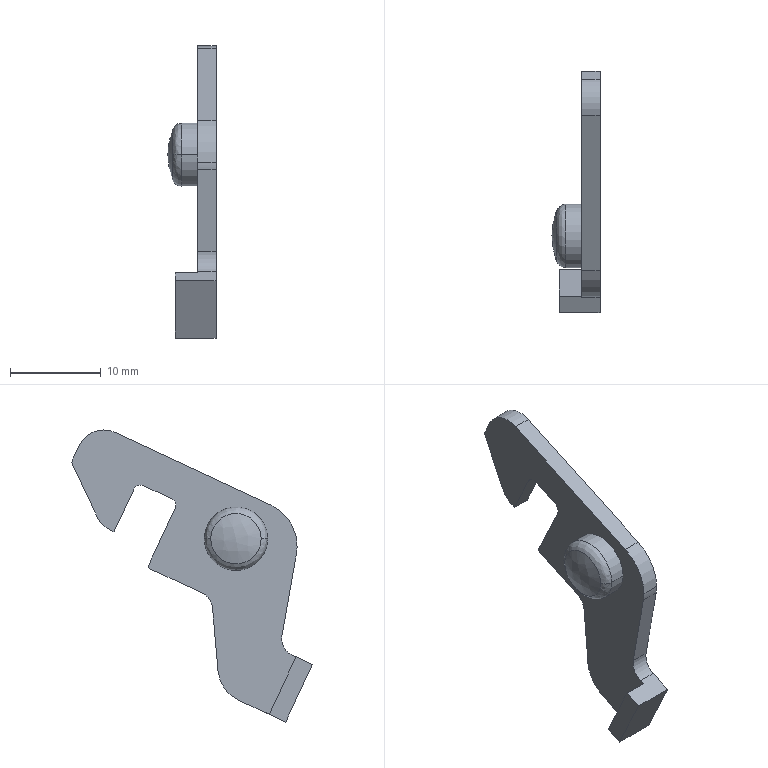Component | SolidWorks | RSDQA32-20DD-M9BL(0_0)-1_RSQ3220(0)-1 | 1 solid | 33 faces | box 5.3 x 26.56 x 32.2 mm | volume 826 mm3 | plane 17 | cylinder 13 | spline 3 | commonest cylinder face diameters 1.6 x3 10 x2 7 x2 6 x2 4 x2 8 x1 0.6 x1
STEP:
#1=COLOUR_RGB('',0.7922,0.8196,0.9333);
#2=FILL_AREA_STYLE_COLOUR('',#1);
#3=FILL_AREA_STYLE('',(#2));
#4=SURFACE_STYLE_FILL_AREA(#3);
#5=SURFACE_SIDE_STYLE('',(#4));
#6=SURFACE_STYLE_USAGE(.BOTH.,#5);
#7=PRESENTATION_STYLE_ASSIGNMENT((#6));
#8=CARTESIAN_POINT('',(0.0703,1.259,-0.6246));
#9=VERTEX_POINT('',#8);
#10=CARTESIAN_POINT('',(0.0703,0.9833,-0.6246));
#11=VERTEX_POINT('',#10);
#12=CARTESIAN_POINT('',(0.0703,1.121,-0.6246));
#13=DIRECTION('',(1.,0.,-0.));
#14=DIRECTION('',(0.,-1.,0.));
#15=AXIS2_PLACEMENT_3D('',#12,#13,#14);
#16=CIRCLE('',#15,0.1378);
#17=EDGE_CURVE('',#9,#11,#16,.T.);
#18=ORIENTED_EDGE('',*,*,#17,.F.);
#19=CARTESIAN_POINT('',(0.0297,1.231,-0.6246));
#20=VERTEX_POINT('',#19);
#21=CARTESIAN_POINT('',(0.0703,1.216,-0.6246));
#22=DIRECTION('',(0.,0.,1.));
#23=DIRECTION('',(0.,1.,0.));
#24=AXIS2_PLACEMENT_3D('',#21,#22,#23);
#25=CIRCLE('',#24,0.04331);
#26=EDGE_CURVE('',#9,#20,#25,.T.);
#27=ORIENTED_EDGE('',*,*,#26,.T.);
#28=CARTESIAN_POINT('',(0.0297,1.012,-0.6246));
#29=VERTEX_POINT('',#28);
#30=CARTESIAN_POINT('',(0.0297,1.121,-0.6246));
#31=DIRECTION('',(1.,0.,-0.));
#32=DIRECTION('',(0.,-1.,0.));
#33=AXIS2_PLACEMENT_3D('',#30,#31,#32);
#34=CIRCLE('',#33,0.1096);
#35=EDGE_CURVE('',#20,#29,#34,.T.);
#36=ORIENTED_EDGE('',*,*,#35,.T.);
#37=CARTESIAN_POINT('',(0.0703,1.027,-0.6246));
#38=DIRECTION('',(-0.,0.,-1.));
#39=DIRECTION('',(0.,-1.,0.));
#40=AXIS2_PLACEMENT_3D('',#37,#38,#39);
#41=CIRCLE('',#40,0.04331);
#42=EDGE_CURVE('',#11,#29,#41,.T.);
#43=ORIENTED_EDGE('',*,*,#42,.F.);
#44=EDGE_LOOP('',(#18,#27,#36,#43));
#45=FACE_OUTER_BOUND('',#44,.T.);
#46=CARTESIAN_POINT('',(0.0703,1.259,-0.6246));
#47=CARTESIAN_POINT('',(0.0703,1.259,-0.349));
#48=CARTESIAN_POINT('',(0.0703,0.9833,-0.349));
#49=CARTESIAN_POINT('',(0.0703,0.9833,-0.6246));
#50=CARTESIAN_POINT('',(0.05158,1.259,-0.6246));
#51=CARTESIAN_POINT('',(0.05158,1.259,-0.349));
#52=CARTESIAN_POINT('',(0.05158,0.9833,-0.349));
#53=CARTESIAN_POINT('',(0.05158,0.9833,-0.6246));
#54=CARTESIAN_POINT('',(0.03621,1.248,-0.6246));
#55=CARTESIAN_POINT('',(0.03621,1.248,-0.3704));
#56=CARTESIAN_POINT('',(0.03621,0.994,-0.3704));
#57=CARTESIAN_POINT('',(0.03621,0.994,-0.6246));
#58=CARTESIAN_POINT('',(0.0297,1.231,-0.6246));
#59=CARTESIAN_POINT('',(0.0297,1.231,-0.4055));
#60=CARTESIAN_POINT('',(0.0297,1.012,-0.4055));
#61=CARTESIAN_POINT('',(0.0297,1.012,-0.6246));
#62=(BOUNDED_SURFACE()B_SPLINE_SURFACE(3,3,((#46,#47,#48,#49),(#50,#51,#52,#53),(#54,#55,#56,#57),(#58,#59,#60,#61)),.UNSPECIFIED.,.F.,.F.,.F.)B_SPLINE_SURFACE_WITH_KNOTS((4,4),(4,4),(0.,1.),(0.,1.),.UNSPECIFIED.)GEOMETRIC_REPRESENTATION_ITEM()RATIONAL_B_SPLINE_SURFACE(((1.,0.3333,0.3333,1.),(0.8806,0.2935,0.2935,0.8806),(0.8806,0.2935,0.2935,0.8806),(1.,0.3333,0.3333,1.)))REPRESENTATION_ITEM('')SURFACE());
#63=ADVANCED_FACE('',(#45),#62,.T.);
#64=CARTESIAN_POINT('',(0.14,0.9696,-0.4781));
#65=VERTEX_POINT('',#64);
#66=CARTESIAN_POINT('',(0.14,0.8559,-0.6565));
#67=VERTEX_POINT('',#66);
#68=CARTESIAN_POINT('',(0.14,1.053,-0.6565));
#69=DIRECTION('',(1.,0.,-0.));
#70=DIRECTION('',(0.,-1.,0.));
#71=AXIS2_PLACEMENT_3D('',#68,#69,#70);
#72=CIRCLE('',#71,0.1969);
#73=EDGE_CURVE('',#65,#67,#72,.T.);
#74=ORIENTED_EDGE('',*,*,#73,.T.);
#75=CARTESIAN_POINT('',(0.2187,0.8559,-0.6565));
#76=VERTEX_POINT('',#75);
#77=CARTESIAN_POINT('',(0.14,0.8559,-0.6565));
#78=DIRECTION('',(1.,0.,-0.));
#79=VECTOR('',#78,39.37);
#80=LINE('',#77,#79);
#81=EDGE_CURVE('',#67,#76,#80,.T.);
#82=ORIENTED_EDGE('',*,*,#81,.T.);
#83=CARTESIAN_POINT('',(0.2187,0.9696,-0.4781));
#84=VERTEX_POINT('',#83);
#85=CARTESIAN_POINT('',(0.2187,1.053,-0.6565));
#86=DIRECTION('',(1.,0.,-0.));
#87=DIRECTION('',(0.,-1.,0.));
#88=AXIS2_PLACEMENT_3D('',#85,#86,#87);
#89=CIRCLE('',#88,0.1969);
#90=EDGE_CURVE('',#84,#76,#89,.T.);
#91=ORIENTED_EDGE('',*,*,#90,.F.);
#92=CARTESIAN_POINT('',(0.14,0.9696,-0.4781));
#93=DIRECTION('',(-1.,-0.,0.));
#94=VECTOR('',#93,39.37);
#95=LINE('',#92,#94);
#96=EDGE_CURVE('',#84,#65,#95,.T.);
#97=ORIENTED_EDGE('',*,*,#96,.T.);
#98=EDGE_LOOP('',(#74,#82,#91,#97));
#99=FACE_OUTER_BOUND('',#98,.T.);
#100=CARTESIAN_POINT('',(0.14,1.053,-0.6565));
#101=DIRECTION('',(1.,0.,-0.));
#102=DIRECTION('',(0.,-1.,0.));
#103=AXIS2_PLACEMENT_3D('',#100,#101,#102);
#104=CYLINDRICAL_SURFACE('',#103,0.1969);
#105=ADVANCED_FACE('',(#99),#104,.T.);
#106=CARTESIAN_POINT('',(0.14,1.385,-0.4927));
#107=VERTEX_POINT('',#106);
#108=CARTESIAN_POINT('',(0.14,1.382,-0.4794));
#109=VERTEX_POINT('',#108);
#110=CARTESIAN_POINT('',(0.14,1.414,-0.4794));
#111=DIRECTION('',(-1.,-0.,0.));
#112=DIRECTION('',(0.,-1.,0.));
#113=AXIS2_PLACEMENT_3D('',#110,#111,#112);
#114=CIRCLE('',#113,0.0315);
#115=EDGE_CURVE('',#107,#109,#114,.T.);
#116=ORIENTED_EDGE('',*,*,#115,.T.);
#117=CARTESIAN_POINT('',(0.2187,1.382,-0.4794));
#118=VERTEX_POINT('',#117);
#119=CARTESIAN_POINT('',(0.14,1.382,-0.4794));
#120=DIRECTION('',(1.,0.,-0.));
#121=VECTOR('',#120,39.37);
#122=LINE('',#119,#121);
#123=EDGE_CURVE('',#109,#118,#122,.T.);
#124=ORIENTED_EDGE('',*,*,#123,.T.);
#125=CARTESIAN_POINT('',(0.2187,1.385,-0.4927));
#126=VERTEX_POINT('',#125);
#127=CARTESIAN_POINT('',(0.2187,1.414,-0.4794));
#128=DIRECTION('',(1.,0.,-0.));
#129=DIRECTION('',(0.,-1.,0.));
#130=AXIS2_PLACEMENT_3D('',#127,#128,#129);
#131=CIRCLE('',#130,0.0315);
#132=EDGE_CURVE('',#118,#126,#131,.T.);
#133=ORIENTED_EDGE('',*,*,#132,.T.);
#134=CARTESIAN_POINT('',(0.14,1.385,-0.4927));
#135=DIRECTION('',(1.,0.,-0.));
#136=VECTOR('',#135,39.37);
#137=LINE('',#134,#136);
#138=EDGE_CURVE('',#107,#126,#137,.T.);
#139=ORIENTED_EDGE('',*,*,#138,.F.);
#140=EDGE_LOOP('',(#116,#124,#133,#139));
#141=FACE_OUTER_BOUND('',#140,.T.);
#142=CARTESIAN_POINT('',(0.14,1.414,-0.4794));
#143=DIRECTION('',(1.,0.,-0.));
#144=DIRECTION('',(0.,-1.,0.));
#145=AXIS2_PLACEMENT_3D('',#142,#143,#144);
#146=CYLINDRICAL_SURFACE('',#145,0.0315);
#147=ADVANCED_FACE('',(#141),#146,.F.);
#148=CARTESIAN_POINT('',(0.0703,1.121,-0.6246));
#149=DIRECTION('',(1.,0.,-0.));
#150=DIRECTION('',(0.,-1.,0.));
#151=AXIS2_PLACEMENT_3D('',#148,#149,#150);
#152=CIRCLE('',#151,0.1378);
#153=EDGE_CURVE('',#11,#9,#152,.T.);
#154=ORIENTED_EDGE('',*,*,#153,.T.);
#155=CARTESIAN_POINT('',(0.14,1.259,-0.6246));
#156=VERTEX_POINT('',#155);
#157=CARTESIAN_POINT('',(0.1051,1.259,-0.6246));
#158=DIRECTION('',(1.,0.,-0.));
#159=VECTOR('',#158,39.37);
#160=LINE('',#157,#159);
#161=EDGE_CURVE('',#9,#156,#160,.T.);
#162=ORIENTED_EDGE('',*,*,#161,.T.);
#163=CARTESIAN_POINT('',(0.14,0.9833,-0.6246));
#164=VERTEX_POINT('',#163);
#165=CARTESIAN_POINT('',(0.14,1.121,-0.6246));
#166=DIRECTION('',(-1.,-0.,0.));
#167=DIRECTION('',(0.,-1.,0.));
#168=AXIS2_PLACEMENT_3D('',#165,#166,#167);
#169=CIRCLE('',#168,0.1378);
#170=EDGE_CURVE('',#156,#164,#169,.T.);
#171=ORIENTED_EDGE('',*,*,#170,.T.);
#172=CARTESIAN_POINT('',(0.1051,0.9833,-0.6246));
#173=DIRECTION('',(1.,0.,-0.));
#174=VECTOR('',#173,39.37);
#175=LINE('',#172,#174);
#176=EDGE_CURVE('',#11,#164,#175,.T.);
#177=ORIENTED_EDGE('',*,*,#176,.F.);
#178=EDGE_LOOP('',(#154,#162,#171,#177));
#179=FACE_OUTER_BOUND('',#178,.T.);
#180=CARTESIAN_POINT('',(0.1051,1.121,-0.6246));
#181=DIRECTION('',(1.,0.,-0.));
#182=DIRECTION('',(0.,-1.,0.));
#183=AXIS2_PLACEMENT_3D('',#180,#181,#182);
#184=CYLINDRICAL_SURFACE('',#183,0.1378);
#185=ADVANCED_FACE('',(#179),#184,.T.);
#186=CARTESIAN_POINT('',(0.2187,1.666,-0.5876));
#187=VERTEX_POINT('',#186);
#188=CARTESIAN_POINT('',(0.2187,1.65,-0.5951));
#189=VERTEX_POINT('',#188);
#190=CARTESIAN_POINT('',(0.2187,1.666,-0.5876));
#191=DIRECTION('',(-0.,-0.9063,-0.4226));
#192=VECTOR('',#191,39.37);
#193=LINE('',#190,#192);
#194=EDGE_CURVE('',#187,#189,#193,.T.);
#195=ORIENTED_EDGE('',*,*,#194,.F.);
#196=CARTESIAN_POINT('',(0.2187,1.723,-0.5305));
#197=VERTEX_POINT('',#196);
#198=CARTESIAN_POINT('',(0.2187,1.616,-0.4806));
#199=DIRECTION('',(1.,0.,-0.));
#200=DIRECTION('',(0.,-1.,0.));
#201=AXIS2_PLACEMENT_3D('',#198,#199,#200);
#202=CIRCLE('',#201,0.1181);
#203=EDGE_CURVE('',#187,#197,#202,.T.);
#204=ORIENTED_EDGE('',*,*,#203,.T.);
#205=CARTESIAN_POINT('',(0.2187,1.835,-0.2918));
#206=VERTEX_POINT('',#205);
#207=CARTESIAN_POINT('',(0.2187,1.723,-0.5305));
#208=DIRECTION('',(0.,0.4226,0.9063));
#209=VECTOR('',#208,39.37);
#210=LINE('',#207,#209);
#211=EDGE_CURVE('',#197,#206,#210,.T.);
#212=ORIENTED_EDGE('',*,*,#211,.T.);
#213=CARTESIAN_POINT('',(0.2187,1.801,-0.2205));
#214=VERTEX_POINT('',#213);
#215=CARTESIAN_POINT('',(0.2187,1.835,-0.2918));
#216=DIRECTION('',(0.,-0.4226,0.9063));
#217=VECTOR('',#216,39.37);
#218=LINE('',#215,#217);
#219=EDGE_CURVE('',#206,#214,#218,.T.);
#220=ORIENTED_EDGE('',*,*,#219,.T.);
#221=CARTESIAN_POINT('',(0.2187,1.644,-0.1634));
#222=VERTEX_POINT('',#221);
#223=CARTESIAN_POINT('',(0.2187,1.694,-0.2704));
#224=DIRECTION('',(1.,0.,-0.));
#225=DIRECTION('',(0.,-1.,0.));
#226=AXIS2_PLACEMENT_3D('',#223,#224,#225);
#227=CIRCLE('',#226,0.1181);
#228=EDGE_CURVE('',#214,#222,#227,.T.);
#229=ORIENTED_EDGE('',*,*,#228,.T.);
#230=CARTESIAN_POINT('',(0.2187,1.644,-0.1634));
#231=DIRECTION('',(-0.,-0.9063,-0.4226));
#232=VECTOR('',#231,39.37);
#233=LINE('',#230,#232);
#234=EDGE_CURVE('',#222,#84,#233,.T.);
#235=ORIENTED_EDGE('',*,*,#234,.T.);
#236=ORIENTED_EDGE('',*,*,#90,.T.);
#237=CARTESIAN_POINT('',(0.2187,0.8589,-0.6907));
#238=VERTEX_POINT('',#237);
#239=CARTESIAN_POINT('',(0.2187,1.053,-0.6565));
#240=DIRECTION('',(1.,0.,-0.));
#241=DIRECTION('',(0.,-1.,0.));
#242=AXIS2_PLACEMENT_3D('',#239,#240,#241);
#243=CIRCLE('',#242,0.1969);
#244=EDGE_CURVE('',#76,#238,#243,.T.);
#245=ORIENTED_EDGE('',*,*,#244,.T.);
#246=CARTESIAN_POINT('',(0.2187,0.9213,-1.044));
#247=VERTEX_POINT('',#246);
#248=CARTESIAN_POINT('',(0.2187,0.8589,-0.6907));
#249=DIRECTION('',(-0.,0.1736,-0.9848));
#250=VECTOR('',#249,39.37);
#251=LINE('',#248,#250);
#252=EDGE_CURVE('',#238,#247,#251,.T.);
#253=ORIENTED_EDGE('',*,*,#252,.T.);
#254=CARTESIAN_POINT('',(0.2187,0.877,-1.129));
#255=VERTEX_POINT('',#254);
#256=CARTESIAN_POINT('',(0.2187,0.8438,-1.058));
#257=DIRECTION('',(-1.,-0.,0.));
#258=DIRECTION('',(0.,-1.,-0.));
#259=AXIS2_PLACEMENT_3D('',#256,#257,#258);
#260=CIRCLE('',#259,0.07874);
#261=EDGE_CURVE('',#247,#255,#260,.T.);
#262=ORIENTED_EDGE('',*,*,#261,.T.);
#263=CARTESIAN_POINT('',(0.2187,0.7891,-1.17));
#264=VERTEX_POINT('',#263);
#265=CARTESIAN_POINT('',(0.2187,0.877,-1.129));
#266=DIRECTION('',(-0.,-0.9063,-0.4226));
#267=VECTOR('',#266,39.37);
#268=LINE('',#265,#267);
#269=EDGE_CURVE('',#255,#264,#268,.T.);
#270=ORIENTED_EDGE('',*,*,#269,.T.);
#271=CARTESIAN_POINT('',(0.2187,0.9056,-1.42));
#272=VERTEX_POINT('',#271);
#273=CARTESIAN_POINT('',(0.2187,0.7891,-1.17));
#274=DIRECTION('',(-0.,0.4226,-0.9063));
#275=VECTOR('',#274,39.37);
#276=LINE('',#273,#275);
#277=EDGE_CURVE('',#264,#272,#276,.T.);
#278=ORIENTED_EDGE('',*,*,#277,.T.);
#279=CARTESIAN_POINT('',(0.2187,1.109,-1.325));
#280=VERTEX_POINT('',#279);
#281=CARTESIAN_POINT('',(0.2187,0.9056,-1.42));
#282=DIRECTION('',(0.,0.9063,0.4226));
#283=VECTOR('',#282,39.37);
#284=LINE('',#281,#283);
#285=EDGE_CURVE('',#272,#280,#284,.T.);
#286=ORIENTED_EDGE('',*,*,#285,.T.);
#287=CARTESIAN_POINT('',(0.2187,1.199,-1.196));
#288=VERTEX_POINT('',#287);
#289=CARTESIAN_POINT('',(0.2187,1.042,-1.183));
#290=DIRECTION('',(1.,0.,-0.));
#291=DIRECTION('',(0.,-1.,0.));
#292=AXIS2_PLACEMENT_3D('',#289,#290,#291);
#293=CIRCLE('',#292,0.1575);
#294=EDGE_CURVE('',#280,#288,#293,.T.);
#295=ORIENTED_EDGE('',*,*,#294,.T.);
#296=CARTESIAN_POINT('',(0.2187,1.223,-0.9247));
#297=VERTEX_POINT('',#296);
#298=CARTESIAN_POINT('',(0.2187,1.199,-1.196));
#299=DIRECTION('',(0.,0.08716,0.9962));
#300=VECTOR('',#299,39.37);
#301=LINE('',#298,#300);
#302=EDGE_CURVE('',#288,#297,#301,.T.);
#303=ORIENTED_EDGE('',*,*,#302,.T.);
#304=CARTESIAN_POINT('',(0.2187,1.268,-0.8602));
#305=VERTEX_POINT('',#304);
#306=CARTESIAN_POINT('',(0.2187,1.301,-0.9316));
#307=DIRECTION('',(-1.,-0.,0.));
#308=DIRECTION('',(0.,-1.,0.));
#309=AXIS2_PLACEMENT_3D('',#306,#307,#308);
#310=CIRCLE('',#309,0.07874);
#311=EDGE_CURVE('',#297,#305,#310,.T.);
#312=ORIENTED_EDGE('',*,*,#311,.T.);
#313=CARTESIAN_POINT('',(0.2187,1.494,-0.7546));
#314=VERTEX_POINT('',#313);
#315=CARTESIAN_POINT('',(0.2187,1.268,-0.8602));
#316=DIRECTION('',(0.,0.9063,0.4226));
#317=VECTOR('',#316,39.37);
#318=LINE('',#315,#317);
#319=EDGE_CURVE('',#305,#314,#318,.T.);
#320=ORIENTED_EDGE('',*,*,#319,.T.);
#321=CARTESIAN_POINT('',(0.2187,1.5,-0.7389));
#322=VERTEX_POINT('',#321);
#323=CARTESIAN_POINT('',(0.2187,1.489,-0.7439));
#324=DIRECTION('',(-1.,-0.,0.));
#325=DIRECTION('',(0.,-1.,0.));
#326=AXIS2_PLACEMENT_3D('',#323,#324,#325);
#327=CIRCLE('',#326,0.01181);
#328=EDGE_CURVE('',#322,#314,#327,.T.);
#329=ORIENTED_EDGE('',*,*,#328,.F.);
#330=CARTESIAN_POINT('',(0.2187,1.5,-0.7389));
#331=DIRECTION('',(0.,-0.4226,0.9063));
#332=VECTOR('',#331,39.37);
#333=LINE('',#330,#332);
#334=EDGE_CURVE('',#322,#126,#333,.T.);
#335=ORIENTED_EDGE('',*,*,#334,.T.);
#336=ORIENTED_EDGE('',*,*,#132,.F.);
#337=CARTESIAN_POINT('',(0.2187,1.401,-0.4509));
#338=VERTEX_POINT('',#337);
#339=CARTESIAN_POINT('',(0.2187,1.414,-0.4794));
#340=DIRECTION('',(1.,0.,-0.));
#341=DIRECTION('',(0.,-1.,0.));
#342=AXIS2_PLACEMENT_3D('',#339,#340,#341);
#343=CIRCLE('',#342,0.0315);
#344=EDGE_CURVE('',#338,#118,#343,.T.);
#345=ORIENTED_EDGE('',*,*,#344,.F.);
#346=CARTESIAN_POINT('',(0.2187,1.522,-0.3943));
#347=VERTEX_POINT('',#346);
#348=CARTESIAN_POINT('',(0.2187,1.401,-0.4509));
#349=DIRECTION('',(0.,0.9063,0.4226));
#350=VECTOR('',#349,39.37);
#351=LINE('',#348,#350);
#352=EDGE_CURVE('',#338,#347,#351,.T.);
#353=ORIENTED_EDGE('',*,*,#352,.T.);
#354=CARTESIAN_POINT('',(0.2187,1.564,-0.4095));
#355=VERTEX_POINT('',#354);
#356=CARTESIAN_POINT('',(0.2187,1.535,-0.4228));
#357=DIRECTION('',(1.,0.,-0.));
#358=DIRECTION('',(0.,-1.,0.));
#359=AXIS2_PLACEMENT_3D('',#356,#357,#358);
#360=CIRCLE('',#359,0.0315);
#361=EDGE_CURVE('',#355,#347,#360,.T.);
#362=ORIENTED_EDGE('',*,*,#361,.F.);
#363=CARTESIAN_POINT('',(0.2187,1.564,-0.4095));
#364=DIRECTION('',(-0.,0.4226,-0.9063));
#365=VECTOR('',#364,39.37);
#366=LINE('',#363,#365);
#367=EDGE_CURVE('',#355,#189,#366,.T.);
#368=ORIENTED_EDGE('',*,*,#367,.T.);
#369=EDGE_LOOP('',(#195,#204,#212,#220,#229,#235,#236,#245,#253,#262,#270,#278,#286,#295,#303,#312,#320,#329,#335,#336,#345,#353,#362,#368));
#370=FACE_OUTER_BOUND('',#369,.T.);
#371=CARTESIAN_POINT('',(0.2187,0.7667,-0.9002));
#372=DIRECTION('',(1.,0.,-0.));
#373=DIRECTION('',(0.,-1.,-0.));
#374=AXIS2_PLACEMENT_3D('',#371,#372,#373);
#375=PLANE('',#374);
#376=ADVANCED_FACE('',(#370),#375,.T.);
#377=CARTESIAN_POINT('',(0.14,1.666,-0.5876));
#378=VERTEX_POINT('',#377);
#379=CARTESIAN_POINT('',(0.14,1.723,-0.5305));
#380=VERTEX_POINT('',#379);
#381=CARTESIAN_POINT('',(0.14,1.616,-0.4806));
#382=DIRECTION('',(1.,0.,-0.));
#383=DIRECTION('',(0.,-1.,0.));
#384=AXIS2_PLACEMENT_3D('',#381,#382,#383);
#385=CIRCLE('',#384,0.1181);
#386=EDGE_CURVE('',#378,#380,#385,.T.);
#387=ORIENTED_EDGE('',*,*,#386,.T.);
#388=CARTESIAN_POINT('',(0.14,1.723,-0.5305));
#389=DIRECTION('',(1.,0.,-0.));
#390=VECTOR('',#389,39.37);
#391=LINE('',#388,#390);
#392=EDGE_CURVE('',#380,#197,#391,.T.);
#393=ORIENTED_EDGE('',*,*,#392,.T.);
#394=ORIENTED_EDGE('',*,*,#203,.F.);
#395=CARTESIAN_POINT('',(0.14,1.666,-0.5876));
#396=DIRECTION('',(-1.,-0.,0.));
#397=VECTOR('',#396,39.37);
#398=LINE('',#395,#397);
#399=EDGE_CURVE('',#187,#378,#398,.T.);
#400=ORIENTED_EDGE('',*,*,#399,.T.);
#401=EDGE_LOOP('',(#387,#393,#394,#400));
#402=FACE_OUTER_BOUND('',#401,.T.);
#403=CARTESIAN_POINT('',(0.14,1.616,-0.4806));
#404=DIRECTION('',(1.,0.,-0.));
#405=DIRECTION('',(0.,-1.,0.));
#406=AXIS2_PLACEMENT_3D('',#403,#404,#405);
#407=CYLINDRICAL_SURFACE('',#406,0.1181);
#408=ADVANCED_FACE('',(#402),#407,.T.);
#409=CARTESIAN_POINT('',(0.14,1.564,-0.4095));
#410=VERTEX_POINT('',#409);
#411=CARTESIAN_POINT('',(0.14,1.65,-0.5951));
#412=VERTEX_POINT('',#411);
#413=CARTESIAN_POINT('',(0.14,1.65,-0.5951));
#414=DIRECTION('',(-0.,0.4226,-0.9063));
#415=VECTOR('',#414,39.37);
#416=LINE('',#413,#415);
#417=EDGE_CURVE('',#410,#412,#416,.T.);
#418=ORIENTED_EDGE('',*,*,#417,.T.);
#419=CARTESIAN_POINT('',(0.14,1.65,-0.5951));
#420=DIRECTION('',(1.,0.,-0.));
#421=VECTOR('',#420,39.37);
#422=LINE('',#419,#421);
#423=EDGE_CURVE('',#412,#189,#422,.T.);
#424=ORIENTED_EDGE('',*,*,#423,.T.);
#425=ORIENTED_EDGE('',*,*,#367,.F.);
#426=CARTESIAN_POINT('',(0.14,1.564,-0.4095));
#427=DIRECTION('',(-1.,-0.,0.));
#428=VECTOR('',#427,39.37);
#429=LINE('',#426,#428);
#430=EDGE_CURVE('',#355,#410,#429,.T.);
#431=ORIENTED_EDGE('',*,*,#430,.T.);
#432=EDGE_LOOP('',(#418,#424,#425,#431));
#433=FACE_OUTER_BOUND('',#432,.T.);
#434=CARTESIAN_POINT('',(0.14,1.65,-0.5951));
#435=DIRECTION('',(-0.,-0.9063,-0.4226));
#436=DIRECTION('',(-0.,0.4226,-0.9063));
#437=AXIS2_PLACEMENT_3D('',#434,#435,#436);
#438=PLANE('',#437);
#439=ADVANCED_FACE('',(#433),#438,.T.);
#440=CARTESIAN_POINT('',(0.14,1.401,-0.4509));
#441=VERTEX_POINT('',#440);
#442=CARTESIAN_POINT('',(0.14,1.522,-0.3943));
#443=VERTEX_POINT('',#442);
#444=CARTESIAN_POINT('',(0.14,1.522,-0.3943));
#445=DIRECTION('',(0.,0.9063,0.4226));
#446=VECTOR('',#445,39.37);
#447=LINE('',#444,#446);
#448=EDGE_CURVE('',#441,#443,#447,.T.);
#449=ORIENTED_EDGE('',*,*,#448,.T.);
#450=CARTESIAN_POINT('',(0.14,1.522,-0.3943));
#451=DIRECTION('',(1.,0.,-0.));
#452=VECTOR('',#451,39.37);
#453=LINE('',#450,#452);
#454=EDGE_CURVE('',#443,#347,#453,.T.);
#455=ORIENTED_EDGE('',*,*,#454,.T.);
#456=ORIENTED_EDGE('',*,*,#352,.F.);
#457=CARTESIAN_POINT('',(0.14,1.401,-0.4509));
#458=DIRECTION('',(-1.,-0.,0.));
#459=VECTOR('',#458,39.37);
#460=LINE('',#457,#459);
#461=EDGE_CURVE('',#338,#441,#460,.T.);
#462=ORIENTED_EDGE('',*,*,#461,.T.);
#463=EDGE_LOOP('',(#449,#455,#456,#462));
#464=FACE_OUTER_BOUND('',#463,.T.);
#465=CARTESIAN_POINT('',(0.14,1.522,-0.3943));
#466=DIRECTION('',(-0.,0.4226,-0.9063));
#467=DIRECTION('',(0.,0.9063,0.4226));
#468=AXIS2_PLACEMENT_3D('',#465,#466,#467);
#469=PLANE('',#468);
#470=ADVANCED_FACE('',(#464),#469,.T.);
#471=CARTESIAN_POINT('',(0.14,1.5,-0.7389));
#472=VERTEX_POINT('',#471);
#473=CARTESIAN_POINT('',(0.14,1.385,-0.4927));
#474=DIRECTION('',(0.,-0.4226,0.9063));
#475=VECTOR('',#474,39.37);
#476=LINE('',#473,#475);
#477=EDGE_CURVE('',#472,#107,#476,.T.);
#478=ORIENTED_EDGE('',*,*,#477,.T.);
#479=ORIENTED_EDGE('',*,*,#138,.T.);
#480=ORIENTED_EDGE('',*,*,#334,.F.);
#481=CARTESIAN_POINT('',(0.14,1.5,-0.7389));
#482=DIRECTION('',(-1.,-0.,0.));
#483=VECTOR('',#482,39.37);
#484=LINE('',#481,#483);
#485=EDGE_CURVE('',#322,#472,#484,.T.);
#486=ORIENTED_EDGE('',*,*,#485,.T.);
#487=EDGE_LOOP('',(#478,#479,#480,#486));
#488=FACE_OUTER_BOUND('',#487,.T.);
#489=CARTESIAN_POINT('',(0.14,1.385,-0.4927));
#490=DIRECTION('',(0.,0.9063,0.4226));
#491=DIRECTION('',(0.,-0.4226,0.9063));
#492=AXIS2_PLACEMENT_3D('',#489,#490,#491);
#493=PLANE('',#492);
#494=ADVANCED_FACE('',(#488),#493,.T.);
#495=CARTESIAN_POINT('',(0.14,1.268,-0.8602));
#496=VERTEX_POINT('',#495);
#497=CARTESIAN_POINT('',(0.14,1.494,-0.7546));
#498=VERTEX_POINT('',#497);
#499=CARTESIAN_POINT('',(0.14,1.494,-0.7546));
#500=DIRECTION('',(0.,0.9063,0.4226));
#501=VECTOR('',#500,39.37);
#502=LINE('',#499,#501);
#503=EDGE_CURVE('',#496,#498,#502,.T.);
#504=ORIENTED_EDGE('',*,*,#503,.T.);
#505=CARTESIAN_POINT('',(0.14,1.494,-0.7546));
#506=DIRECTION('',(1.,0.,-0.));
#507=VECTOR('',#506,39.37);
#508=LINE('',#505,#507);
#509=EDGE_CURVE('',#498,#314,#508,.T.);
#510=ORIENTED_EDGE('',*,*,#509,.T.);
#511=ORIENTED_EDGE('',*,*,#319,.F.);
#512=CARTESIAN_POINT('',(0.14,1.268,-0.8602));
#513=DIRECTION('',(-1.,-0.,0.));
#514=VECTOR('',#513,39.37);
#515=LINE('',#512,#514);
#516=EDGE_CURVE('',#305,#496,#515,.T.);
#517=ORIENTED_EDGE('',*,*,#516,.T.);
#518=EDGE_LOOP('',(#504,#510,#511,#517));
#519=FACE_OUTER_BOUND('',#518,.T.);
#520=CARTESIAN_POINT('',(0.14,1.494,-0.7546));
#521=DIRECTION('',(-0.,0.4226,-0.9063));
#522=DIRECTION('',(0.,0.9063,0.4226));
#523=AXIS2_PLACEMENT_3D('',#520,#521,#522);
#524=PLANE('',#523);
#525=ADVANCED_FACE('',(#519),#524,.T.);
#526=CARTESIAN_POINT('',(0.14,1.223,-0.9247));
#527=VERTEX_POINT('',#526);
#528=CARTESIAN_POINT('',(0.14,1.301,-0.9316));
#529=DIRECTION('',(-1.,-0.,0.));
#530=DIRECTION('',(0.,-1.,0.));
#531=AXIS2_PLACEMENT_3D('',#528,#529,#530);
#532=CIRCLE('',#531,0.07874);
#533=EDGE_CURVE('',#527,#496,#532,.T.);
#534=ORIENTED_EDGE('',*,*,#533,.T.);
#535=ORIENTED_EDGE('',*,*,#516,.F.);
#536=ORIENTED_EDGE('',*,*,#311,.F.);
#537=CARTESIAN_POINT('',(0.14,1.223,-0.9247));
#538=DIRECTION('',(-1.,-0.,0.));
#539=VECTOR('',#538,39.37);
#540=LINE('',#537,#539);
#541=EDGE_CURVE('',#297,#527,#540,.T.);
#542=ORIENTED_EDGE('',*,*,#541,.T.);
#543=EDGE_LOOP('',(#534,#535,#536,#542));
#544=FACE_OUTER_BOUND('',#543,.T.);
#545=CARTESIAN_POINT('',(0.14,1.301,-0.9316));
#546=DIRECTION('',(1.,0.,-0.));
#547=DIRECTION('',(0.,-1.,0.));
#548=AXIS2_PLACEMENT_3D('',#545,#546,#547);
#549=CYLINDRICAL_SURFACE('',#548,0.07874);
#550=ADVANCED_FACE('',(#544),#549,.F.);
#551=CARTESIAN_POINT('',(0.14,1.199,-1.196));
#552=VERTEX_POINT('',#551);
#553=CARTESIAN_POINT('',(0.14,1.223,-0.9247));
#554=DIRECTION('',(0.,0.08716,0.9962));
#555=VECTOR('',#554,39.37);
#556=LINE('',#553,#555);
#557=EDGE_CURVE('',#552,#527,#556,.T.);
#558=ORIENTED_EDGE('',*,*,#557,.T.);
#559=ORIENTED_EDGE('',*,*,#541,.F.);
#560=ORIENTED_EDGE('',*,*,#302,.F.);
#561=CARTESIAN_POINT('',(0.14,1.199,-1.196));
#562=DIRECTION('',(-1.,-0.,0.));
#563=VECTOR('',#562,39.37);
#564=LINE('',#561,#563);
#565=EDGE_CURVE('',#288,#552,#564,.T.);
#566=ORIENTED_EDGE('',*,*,#565,.T.);
#567=EDGE_LOOP('',(#558,#559,#560,#566));
#568=FACE_OUTER_BOUND('',#567,.T.);
#569=CARTESIAN_POINT('',(0.14,1.223,-0.9247));
#570=DIRECTION('',(-0.,0.9962,-0.08716));
#571=DIRECTION('',(0.,0.08716,0.9962));
#572=AXIS2_PLACEMENT_3D('',#569,#570,#571);
#573=PLANE('',#572);
#574=ADVANCED_FACE('',(#568),#573,.T.);
#575=CARTESIAN_POINT('',(0.14,1.109,-1.325));
#576=VERTEX_POINT('',#575);
#577=CARTESIAN_POINT('',(0.14,1.042,-1.183));
#578=DIRECTION('',(1.,0.,-0.));
#579=DIRECTION('',(0.,-1.,0.));
#580=AXIS2_PLACEMENT_3D('',#577,#578,#579);
#581=CIRCLE('',#580,0.1575);
#582=EDGE_CURVE('',#576,#552,#581,.T.);
#583=ORIENTED_EDGE('',*,*,#582,.T.);
#584=ORIENTED_EDGE('',*,*,#565,.F.);
#585=ORIENTED_EDGE('',*,*,#294,.F.);
#586=CARTESIAN_POINT('',(0.14,1.109,-1.325));
#587=DIRECTION('',(-1.,-0.,0.));
#588=VECTOR('',#587,39.37);
#589=LINE('',#586,#588);
#590=EDGE_CURVE('',#280,#576,#589,.T.);
#591=ORIENTED_EDGE('',*,*,#590,.T.);
#592=EDGE_LOOP('',(#583,#584,#585,#591));
#593=FACE_OUTER_BOUND('',#592,.T.);
#594=CARTESIAN_POINT('',(0.14,1.042,-1.183));
#595=DIRECTION('',(1.,0.,-0.));
#596=DIRECTION('',(0.,-1.,0.));
#597=AXIS2_PLACEMENT_3D('',#594,#595,#596);
#598=CYLINDRICAL_SURFACE('',#597,0.1575);
#599=ADVANCED_FACE('',(#593),#598,.T.);
#600=CARTESIAN_POINT('',(0.14,0.9769,-1.387));
#601=VERTEX_POINT('',#600);
#602=CARTESIAN_POINT('',(0.14,1.109,-1.325));
#603=DIRECTION('',(0.,0.9063,0.4226));
#604=VECTOR('',#603,39.37);
#605=LINE('',#602,#604);
#606=EDGE_CURVE('',#601,#576,#605,.T.);
#607=ORIENTED_EDGE('',*,*,#606,.T.);
#608=ORIENTED_EDGE('',*,*,#590,.F.);
#609=ORIENTED_EDGE('',*,*,#285,.F.);
#610=CARTESIAN_POINT('',(0.04153,0.9056,-1.42));
#611=VERTEX_POINT('',#610);
#612=CARTESIAN_POINT('',(0.14,0.9056,-1.42));
#613=DIRECTION('',(-1.,-0.,0.));
#614=VECTOR('',#613,39.37);
#615=LINE('',#612,#614);
#616=EDGE_CURVE('',#272,#611,#615,.T.);
#617=ORIENTED_EDGE('',*,*,#616,.T.);
#618=CARTESIAN_POINT('',(0.04153,0.9769,-1.387));
#619=VERTEX_POINT('',#618);
#620=CARTESIAN_POINT('',(0.04153,1.109,-1.325));
#621=DIRECTION('',(0.,0.9063,0.4226));
#622=VECTOR('',#621,39.37);
#623=LINE('',#620,#622);
#624=EDGE_CURVE('',#611,#619,#623,.T.);
#625=ORIENTED_EDGE('',*,*,#624,.T.);
#626=CARTESIAN_POINT('',(0.14,0.9769,-1.387));
#627=DIRECTION('',(1.,0.,-0.));
#628=VECTOR('',#627,39.37);
#629=LINE('',#626,#628);
#630=EDGE_CURVE('',#619,#601,#629,.T.);
#631=ORIENTED_EDGE('',*,*,#630,.T.);
#632=EDGE_LOOP('',(#607,#608,#609,#617,#625,#631));
#633=FACE_OUTER_BOUND('',#632,.T.);
#634=CARTESIAN_POINT('',(0.14,1.109,-1.325));
#635=DIRECTION('',(-0.,0.4226,-0.9063));
#636=DIRECTION('',(0.,0.9063,0.4226));
#637=AXIS2_PLACEMENT_3D('',#634,#635,#636);
#638=PLANE('',#637);
#639=ADVANCED_FACE('',(#633),#638,.T.);
#640=CARTESIAN_POINT('',(0.04153,0.7891,-1.17));
#641=VERTEX_POINT('',#640);
#642=CARTESIAN_POINT('',(0.04153,0.9056,-1.42));
#643=DIRECTION('',(-0.,0.4226,-0.9063));
#644=VECTOR('',#643,39.37);
#645=LINE('',#642,#644);
#646=EDGE_CURVE('',#641,#611,#645,.T.);
#647=ORIENTED_EDGE('',*,*,#646,.T.);
#648=ORIENTED_EDGE('',*,*,#616,.F.);
#649=ORIENTED_EDGE('',*,*,#277,.F.);
#650=CARTESIAN_POINT('',(0.14,0.7891,-1.17));
#651=DIRECTION('',(-1.,-0.,0.));
#652=VECTOR('',#651,39.37);
#653=LINE('',#650,#652);
#654=EDGE_CURVE('',#264,#641,#653,.T.);
#655=ORIENTED_EDGE('',*,*,#654,.T.);
#656=EDGE_LOOP('',(#647,#648,#649,#655));
#657=FACE_OUTER_BOUND('',#656,.T.);
#658=CARTESIAN_POINT('',(0.14,0.9056,-1.42));
#659=DIRECTION('',(-0.,-0.9063,-0.4226));
#660=DIRECTION('',(-0.,0.4226,-0.9063));
#661=AXIS2_PLACEMENT_3D('',#658,#659,#660);
#662=PLANE('',#661);
#663=ADVANCED_FACE('',(#657),#662,.T.);
#664=CARTESIAN_POINT('',(0.04153,0.8605,-1.137));
#665=VERTEX_POINT('',#664);
#666=CARTESIAN_POINT('',(0.04153,0.7891,-1.17));
#667=DIRECTION('',(-0.,-0.9063,-0.4226));
#668=VECTOR('',#667,39.37);
#669=LINE('',#666,#668);
#670=EDGE_CURVE('',#665,#641,#669,.T.);
#671=ORIENTED_EDGE('',*,*,#670,.T.);
#672=ORIENTED_EDGE('',*,*,#654,.F.);
#673=ORIENTED_EDGE('',*,*,#269,.F.);
#674=CARTESIAN_POINT('',(0.14,0.877,-1.129));
#675=VERTEX_POINT('',#674);
#676=CARTESIAN_POINT('',(0.14,0.877,-1.129));
#677=DIRECTION('',(-1.,-0.,0.));
#678=VECTOR('',#677,39.37);
#679=LINE('',#676,#678);
#680=EDGE_CURVE('',#255,#675,#679,.T.);
#681=ORIENTED_EDGE('',*,*,#680,.T.);
#682=CARTESIAN_POINT('',(0.14,0.8605,-1.137));
#683=VERTEX_POINT('',#682);
#684=CARTESIAN_POINT('',(0.14,0.7891,-1.17));
#685=DIRECTION('',(-0.,-0.9063,-0.4226));
#686=VECTOR('',#685,39.37);
#687=LINE('',#684,#686);
#688=EDGE_CURVE('',#675,#683,#687,.T.);
#689=ORIENTED_EDGE('',*,*,#688,.T.);
#690=CARTESIAN_POINT('',(0.14,0.8605,-1.137));
#691=DIRECTION('',(-1.,-0.,0.));
#692=VECTOR('',#691,39.37);
#693=LINE('',#690,#692);
#694=EDGE_CURVE('',#683,#665,#693,.T.);
#695=ORIENTED_EDGE('',*,*,#694,.T.);
#696=EDGE_LOOP('',(#671,#672,#673,#681,#689,#695));
#697=FACE_OUTER_BOUND('',#696,.T.);
#698=CARTESIAN_POINT('',(0.14,0.7891,-1.17));
#699=DIRECTION('',(0.,-0.4226,0.9063));
#700=DIRECTION('',(-0.,-0.9063,-0.4226));
#701=AXIS2_PLACEMENT_3D('',#698,#699,#700);
#702=PLANE('',#701);
#703=ADVANCED_FACE('',(#697),#702,.T.);
#704=CARTESIAN_POINT('',(0.14,0.9213,-1.044));
#705=VERTEX_POINT('',#704);
#706=CARTESIAN_POINT('',(0.14,0.8438,-1.058));
#707=DIRECTION('',(-1.,-0.,0.));
#708=DIRECTION('',(0.,-1.,0.));
#709=AXIS2_PLACEMENT_3D('',#706,#707,#708);
#710=CIRCLE('',#709,0.07874);
#711=EDGE_CURVE('',#705,#675,#710,.T.);
#712=ORIENTED_EDGE('',*,*,#711,.T.);
#713=ORIENTED_EDGE('',*,*,#680,.F.);
#714=ORIENTED_EDGE('',*,*,#261,.F.);
#715=CARTESIAN_POINT('',(0.14,0.9213,-1.044));
#716=DIRECTION('',(-1.,-0.,0.));
#717=VECTOR('',#716,39.37);
#718=LINE('',#715,#717);
#719=EDGE_CURVE('',#247,#705,#718,.T.);
#720=ORIENTED_EDGE('',*,*,#719,.T.);
#721=EDGE_LOOP('',(#712,#713,#714,#720));
#722=FACE_OUTER_BOUND('',#721,.T.);
#723=CARTESIAN_POINT('',(0.14,0.8438,-1.058));
#724=DIRECTION('',(1.,0.,-0.));
#725=DIRECTION('',(0.,-1.,0.));
#726=AXIS2_PLACEMENT_3D('',#723,#724,#725);
#727=CYLINDRICAL_SURFACE('',#726,0.07874);
#728=ADVANCED_FACE('',(#722),#727,.F.);
#729=CARTESIAN_POINT('',(0.14,0.8589,-0.6907));
#730=VERTEX_POINT('',#729);
#731=CARTESIAN_POINT('',(0.14,0.9213,-1.044));
#732=DIRECTION('',(-0.,0.1736,-0.9848));
#733=VECTOR('',#732,39.37);
#734=LINE('',#731,#733);
#735=EDGE_CURVE('',#730,#705,#734,.T.);
#736=ORIENTED_EDGE('',*,*,#735,.T.);
#737=ORIENTED_EDGE('',*,*,#719,.F.);
#738=ORIENTED_EDGE('',*,*,#252,.F.);
#739=CARTESIAN_POINT('',(0.14,0.8589,-0.6907));
#740=DIRECTION('',(-1.,-0.,0.));
#741=VECTOR('',#740,39.37);
#742=LINE('',#739,#741);
#743=EDGE_CURVE('',#238,#730,#742,.T.);
#744=ORIENTED_EDGE('',*,*,#743,.T.);
#745=EDGE_LOOP('',(#736,#737,#738,#744));
#746=FACE_OUTER_BOUND('',#745,.T.);
#747=CARTESIAN_POINT('',(0.14,0.9213,-1.044));
#748=DIRECTION('',(0.,-0.9848,-0.1736));
#749=DIRECTION('',(-0.,0.1736,-0.9848));
#750=AXIS2_PLACEMENT_3D('',#747,#748,#749);
#751=PLANE('',#750);
#752=ADVANCED_FACE('',(#746),#751,.T.);
#753=ORIENTED_EDGE('',*,*,#81,.F.);
#754=CARTESIAN_POINT('',(0.14,1.053,-0.6565));
#755=DIRECTION('',(1.,0.,-0.));
#756=DIRECTION('',(0.,-1.,0.));
#757=AXIS2_PLACEMENT_3D('',#754,#755,#756);
#758=CIRCLE('',#757,0.1969);
#759=EDGE_CURVE('',#67,#730,#758,.T.);
#760=ORIENTED_EDGE('',*,*,#759,.T.);
#761=ORIENTED_EDGE('',*,*,#743,.F.);
#762=ORIENTED_EDGE('',*,*,#244,.F.);
#763=EDGE_LOOP('',(#753,#760,#761,#762));
#764=FACE_OUTER_BOUND('',#763,.T.);
#765=CARTESIAN_POINT('',(0.14,1.053,-0.6565));
#766=DIRECTION('',(1.,0.,-0.));
#767=DIRECTION('',(0.,-1.,0.));
#768=AXIS2_PLACEMENT_3D('',#765,#766,#767);
#769=CYLINDRICAL_SURFACE('',#768,0.1969);
#770=ADVANCED_FACE('',(#764),#769,.T.);
#771=CARTESIAN_POINT('',(0.14,1.644,-0.1634));
#772=VERTEX_POINT('',#771);
#773=CARTESIAN_POINT('',(0.14,0.9696,-0.4781));
#774=DIRECTION('',(-0.,-0.9063,-0.4226));
#775=VECTOR('',#774,39.37);
#776=LINE('',#773,#775);
#777=EDGE_CURVE('',#772,#65,#776,.T.);
#778=ORIENTED_EDGE('',*,*,#777,.T.);
#779=ORIENTED_EDGE('',*,*,#96,.F.);
#780=ORIENTED_EDGE('',*,*,#234,.F.);
#781=CARTESIAN_POINT('',(0.14,1.644,-0.1634));
#782=DIRECTION('',(-1.,-0.,0.));
#783=VECTOR('',#782,39.37);
#784=LINE('',#781,#783);
#785=EDGE_CURVE('',#222,#772,#784,.T.);
#786=ORIENTED_EDGE('',*,*,#785,.T.);
#787=EDGE_LOOP('',(#778,#779,#780,#786));
#788=FACE_OUTER_BOUND('',#787,.T.);
#789=CARTESIAN_POINT('',(0.14,0.9696,-0.4781));
#790=DIRECTION('',(0.,-0.4226,0.9063));
#791=DIRECTION('',(-0.,-0.9063,-0.4226));
#792=AXIS2_PLACEMENT_3D('',#789,#790,#791);
#793=PLANE('',#792);
#794=ADVANCED_FACE('',(#788),#793,.T.);
#795=CARTESIAN_POINT('',(0.14,1.801,-0.2205));
#796=VERTEX_POINT('',#795);
#797=CARTESIAN_POINT('',(0.14,1.694,-0.2704));
#798=DIRECTION('',(1.,0.,-0.));
#799=DIRECTION('',(0.,-1.,0.));
#800=AXIS2_PLACEMENT_3D('',#797,#798,#799);
#801=CIRCLE('',#800,0.1181);
#802=EDGE_CURVE('',#796,#772,#801,.T.);
#803=ORIENTED_EDGE('',*,*,#802,.T.);
#804=ORIENTED_EDGE('',*,*,#785,.F.);
#805=ORIENTED_EDGE('',*,*,#228,.F.);
#806=CARTESIAN_POINT('',(0.14,1.801,-0.2205));
#807=DIRECTION('',(-1.,-0.,0.));
#808=VECTOR('',#807,39.37);
#809=LINE('',#806,#808);
#810=EDGE_CURVE('',#214,#796,#809,.T.);
#811=ORIENTED_EDGE('',*,*,#810,.T.);
#812=EDGE_LOOP('',(#803,#804,#805,#811));
#813=FACE_OUTER_BOUND('',#812,.T.);
#814=CARTESIAN_POINT('',(0.14,1.694,-0.2704));
#815=DIRECTION('',(1.,0.,-0.));
#816=DIRECTION('',(0.,-1.,0.));
#817=AXIS2_PLACEMENT_3D('',#814,#815,#816);
#818=CYLINDRICAL_SURFACE('',#817,0.1181);
#819=ADVANCED_FACE('',(#813),#818,.T.);
#820=CARTESIAN_POINT('',(0.14,1.835,-0.2918));
#821=VERTEX_POINT('',#820);
#822=CARTESIAN_POINT('',(0.14,1.801,-0.2205));
#823=DIRECTION('',(0.,-0.4226,0.9063));
#824=VECTOR('',#823,39.37);
#825=LINE('',#822,#824);
#826=EDGE_CURVE('',#821,#796,#825,.T.);
#827=ORIENTED_EDGE('',*,*,#826,.T.);
#828=ORIENTED_EDGE('',*,*,#810,.F.);
#829=ORIENTED_EDGE('',*,*,#219,.F.);
#830=CARTESIAN_POINT('',(0.14,1.835,-0.2918));
#831=DIRECTION('',(-1.,-0.,0.));
#832=VECTOR('',#831,39.37);
#833=LINE('',#830,#832);
#834=EDGE_CURVE('',#206,#821,#833,.T.);
#835=ORIENTED_EDGE('',*,*,#834,.T.);
#836=EDGE_LOOP('',(#827,#828,#829,#835));
#837=FACE_OUTER_BOUND('',#836,.T.);
#838=CARTESIAN_POINT('',(0.14,1.801,-0.2205));
#839=DIRECTION('',(0.,0.9063,0.4226));
#840=DIRECTION('',(0.,-0.4226,0.9063));
#841=AXIS2_PLACEMENT_3D('',#838,#839,#840);
#842=PLANE('',#841);
#843=ADVANCED_FACE('',(#837),#842,.T.);
#844=CARTESIAN_POINT('',(0.14,1.835,-0.2918));
#845=DIRECTION('',(0.,0.4226,0.9063));
#846=VECTOR('',#845,39.37);
#847=LINE('',#844,#846);
#848=EDGE_CURVE('',#380,#821,#847,.T.);
#849=ORIENTED_EDGE('',*,*,#848,.T.);
#850=ORIENTED_EDGE('',*,*,#834,.F.);
#851=ORIENTED_EDGE('',*,*,#211,.F.);
#852=ORIENTED_EDGE('',*,*,#392,.F.);
#853=EDGE_LOOP('',(#849,#850,#851,#852));
#854=FACE_OUTER_BOUND('',#853,.T.);
#855=CARTESIAN_POINT('',(0.14,1.835,-0.2918));
#856=DIRECTION('',(-0.,0.9063,-0.4226));
#857=DIRECTION('',(0.,0.4226,0.9063));
#858=AXIS2_PLACEMENT_3D('',#855,#856,#857);
#859=PLANE('',#858);
#860=ADVANCED_FACE('',(#854),#859,.T.);
#861=ORIENTED_EDGE('',*,*,#688,.F.);
#862=ORIENTED_EDGE('',*,*,#711,.F.);
#863=ORIENTED_EDGE('',*,*,#735,.F.);
#864=ORIENTED_EDGE('',*,*,#759,.F.);
#865=ORIENTED_EDGE('',*,*,#73,.F.);
#866=ORIENTED_EDGE('',*,*,#777,.F.);
#867=ORIENTED_EDGE('',*,*,#802,.F.);
#868=ORIENTED_EDGE('',*,*,#826,.F.);
#869=ORIENTED_EDGE('',*,*,#848,.F.);
#870=ORIENTED_EDGE('',*,*,#386,.F.);
#871=CARTESIAN_POINT('',(0.14,1.65,-0.5951));
#872=DIRECTION('',(0.,0.9063,0.4226));
#873=VECTOR('',#872,39.37);
#874=LINE('',#871,#873);
#875=EDGE_CURVE('',#412,#378,#874,.T.);
#876=ORIENTED_EDGE('',*,*,#875,.F.);
#877=ORIENTED_EDGE('',*,*,#417,.F.);
#878=CARTESIAN_POINT('',(0.14,1.535,-0.4228));
#879=DIRECTION('',(-1.,-0.,0.));
#880=DIRECTION('',(0.,-1.,-0.));
#881=AXIS2_PLACEMENT_3D('',#878,#879,#880);
#882=CIRCLE('',#881,0.0315);
#883=EDGE_CURVE('',#443,#410,#882,.T.);
#884=ORIENTED_EDGE('',*,*,#883,.F.);
#885=ORIENTED_EDGE('',*,*,#448,.F.);
#886=CARTESIAN_POINT('',(0.14,1.414,-0.4794));
#887=DIRECTION('',(-1.,-0.,0.));
#888=DIRECTION('',(0.,-1.,0.));
#889=AXIS2_PLACEMENT_3D('',#886,#887,#888);
#890=CIRCLE('',#889,0.0315);
#891=EDGE_CURVE('',#109,#441,#890,.T.);
#892=ORIENTED_EDGE('',*,*,#891,.F.);
#893=ORIENTED_EDGE('',*,*,#115,.F.);
#894=ORIENTED_EDGE('',*,*,#477,.F.);
#895=CARTESIAN_POINT('',(0.14,1.489,-0.7439));
#896=DIRECTION('',(1.,0.,-0.));
#897=DIRECTION('',(0.,-1.,0.));
#898=AXIS2_PLACEMENT_3D('',#895,#896,#897);
#899=CIRCLE('',#898,0.01181);
#900=EDGE_CURVE('',#498,#472,#899,.T.);
#901=ORIENTED_EDGE('',*,*,#900,.F.);
#902=ORIENTED_EDGE('',*,*,#503,.F.);
#903=ORIENTED_EDGE('',*,*,#533,.F.);
#904=ORIENTED_EDGE('',*,*,#557,.F.);
#905=ORIENTED_EDGE('',*,*,#582,.F.);
#906=ORIENTED_EDGE('',*,*,#606,.F.);
#907=CARTESIAN_POINT('',(0.14,0.8605,-1.137));
#908=DIRECTION('',(-0.,0.4226,-0.9063));
#909=VECTOR('',#908,39.37);
#910=LINE('',#907,#909);
#911=EDGE_CURVE('',#683,#601,#910,.T.);
#912=ORIENTED_EDGE('',*,*,#911,.F.);
#913=EDGE_LOOP('',(#861,#862,#863,#864,#865,#866,#867,#868,#869,#870,#876,#877,#884,#885,#892,#893,#894,#901,#902,#903,#904,#905,#906,#912));
#914=FACE_OUTER_BOUND('',#913,.T.);
#915=CARTESIAN_POINT('',(0.14,1.121,-0.6246));
#916=DIRECTION('',(-1.,-0.,0.));
#917=DIRECTION('',(0.,-1.,0.));
#918=AXIS2_PLACEMENT_3D('',#915,#916,#917);
#919=CIRCLE('',#918,0.1378);
#920=EDGE_CURVE('',#164,#156,#919,.T.);
#921=ORIENTED_EDGE('',*,*,#920,.F.);
#922=ORIENTED_EDGE('',*,*,#170,.F.);
#923=EDGE_LOOP('',(#921,#922));
#924=FACE_BOUND('',#923,.T.);
#925=CARTESIAN_POINT('',(0.14,0.7667,-0.9002));
#926=DIRECTION('',(1.,0.,-0.));
#927=DIRECTION('',(0.,-1.,-0.));
#928=AXIS2_PLACEMENT_3D('',#925,#926,#927);
#929=PLANE('',#928);
#930=ADVANCED_FACE('',(#914,#924),#929,.F.);
#931=ORIENTED_EDGE('',*,*,#875,.T.);
#932=ORIENTED_EDGE('',*,*,#399,.F.);
#933=ORIENTED_EDGE('',*,*,#194,.T.);
#934=ORIENTED_EDGE('',*,*,#423,.F.);
#935=EDGE_LOOP('',(#931,#932,#933,#934));
#936=FACE_OUTER_BOUND('',#935,.T.);
#937=CARTESIAN_POINT('',(0.14,1.666,-0.5876));
#938=DIRECTION('',(-0.,0.4226,-0.9063));
#939=DIRECTION('',(0.,0.9063,0.4226));
#940=AXIS2_PLACEMENT_3D('',#937,#938,#939);
#941=PLANE('',#940);
#942=ADVANCED_FACE('',(#936),#941,.T.);
#943=ORIENTED_EDGE('',*,*,#883,.T.);
#944=ORIENTED_EDGE('',*,*,#430,.F.);
#945=ORIENTED_EDGE('',*,*,#361,.T.);
#946=ORIENTED_EDGE('',*,*,#454,.F.);
#947=EDGE_LOOP('',(#943,#944,#945,#946));
#948=FACE_OUTER_BOUND('',#947,.T.);
#949=CARTESIAN_POINT('',(0.14,1.535,-0.4228));
#950=DIRECTION('',(1.,0.,-0.));
#951=DIRECTION('',(0.,-1.,0.));
#952=AXIS2_PLACEMENT_3D('',#949,#950,#951);
#953=CYLINDRICAL_SURFACE('',#952,0.0315);
#954=ADVANCED_FACE('',(#948),#953,.F.);
#955=ORIENTED_EDGE('',*,*,#123,.F.);
#956=ORIENTED_EDGE('',*,*,#891,.T.);
#957=ORIENTED_EDGE('',*,*,#461,.F.);
#958=ORIENTED_EDGE('',*,*,#344,.T.);
#959=EDGE_LOOP('',(#955,#956,#957,#958));
#960=FACE_OUTER_BOUND('',#959,.T.);
#961=CARTESIAN_POINT('',(0.14,1.414,-0.4794));
#962=DIRECTION('',(1.,0.,-0.));
#963=DIRECTION('',(0.,-1.,0.));
#964=AXIS2_PLACEMENT_3D('',#961,#962,#963);
#965=CYLINDRICAL_SURFACE('',#964,0.0315);
#966=ADVANCED_FACE('',(#960),#965,.F.);
#967=ORIENTED_EDGE('',*,*,#900,.T.);
#968=ORIENTED_EDGE('',*,*,#485,.F.);
#969=ORIENTED_EDGE('',*,*,#328,.T.);
#970=ORIENTED_EDGE('',*,*,#509,.F.);
#971=EDGE_LOOP('',(#967,#968,#969,#970));
#972=FACE_OUTER_BOUND('',#971,.T.);
#973=CARTESIAN_POINT('',(0.14,1.489,-0.7439));
#974=DIRECTION('',(1.,0.,-0.));
#975=DIRECTION('',(0.,-1.,0.));
#976=AXIS2_PLACEMENT_3D('',#973,#974,#975);
#977=CYLINDRICAL_SURFACE('',#976,0.01181);
#978=ADVANCED_FACE('',(#972),#977,.T.);
#979=ORIENTED_EDGE('',*,*,#911,.T.);
#980=ORIENTED_EDGE('',*,*,#630,.F.);
#981=CARTESIAN_POINT('',(0.04153,0.9769,-1.387));
#982=DIRECTION('',(0.,-0.4226,0.9063));
#983=VECTOR('',#982,39.37);
#984=LINE('',#981,#983);
#985=EDGE_CURVE('',#619,#665,#984,.T.);
#986=ORIENTED_EDGE('',*,*,#985,.T.);
#987=ORIENTED_EDGE('',*,*,#694,.F.);
#988=EDGE_LOOP('',(#979,#980,#986,#987));
#989=FACE_OUTER_BOUND('',#988,.T.);
#990=CARTESIAN_POINT('',(0.14,0.9769,-1.387));
#991=DIRECTION('',(0.,0.9063,0.4226));
#992=DIRECTION('',(0.,-0.4226,0.9063));
#993=AXIS2_PLACEMENT_3D('',#990,#991,#992);
#994=PLANE('',#993);
#995=ADVANCED_FACE('',(#989),#994,.T.);
#996=ORIENTED_EDGE('',*,*,#985,.F.);
#997=ORIENTED_EDGE('',*,*,#624,.F.);
#998=ORIENTED_EDGE('',*,*,#646,.F.);
#999=ORIENTED_EDGE('',*,*,#670,.F.);
#1000=EDGE_LOOP('',(#996,#997,#998,#999));
#1001=FACE_OUTER_BOUND('',#1000,.T.);
#1002=CARTESIAN_POINT('',(0.04153,0.7667,-0.9002));
#1003=DIRECTION('',(1.,0.,-0.));
#1004=DIRECTION('',(0.,-1.,-0.));
#1005=AXIS2_PLACEMENT_3D('',#1002,#1003,#1004);
#1006=PLANE('',#1005);
#1007=ADVANCED_FACE('',(#1001),#1006,.F.);
#1008=ORIENTED_EDGE('',*,*,#161,.F.);
#1009=ORIENTED_EDGE('',*,*,#17,.T.);
#1010=ORIENTED_EDGE('',*,*,#176,.T.);
#1011=ORIENTED_EDGE('',*,*,#920,.T.);
#1012=EDGE_LOOP('',(#1008,#1009,#1010,#1011));
#1013=FACE_OUTER_BOUND('',#1012,.T.);
#1014=CARTESIAN_POINT('',(0.1051,1.121,-0.6246));
#1015=DIRECTION('',(1.,0.,-0.));
#1016=DIRECTION('',(0.,-1.,0.));
#1017=AXIS2_PLACEMENT_3D('',#1014,#1015,#1016);
#1018=CYLINDRICAL_SURFACE('',#1017,0.1378);
#1019=ADVANCED_FACE('',(#1013),#1018,.T.);
#1020=ORIENTED_EDGE('',*,*,#26,.F.);
#1021=ORIENTED_EDGE('',*,*,#153,.F.);
#1022=ORIENTED_EDGE('',*,*,#42,.T.);
#1023=CARTESIAN_POINT('',(0.0297,1.121,-0.6246));
#1024=DIRECTION('',(1.,0.,-0.));
#1025=DIRECTION('',(0.,-1.,0.));
#1026=AXIS2_PLACEMENT_3D('',#1023,#1024,#1025);
#1027=CIRCLE('',#1026,0.1096);
#1028=EDGE_CURVE('',#29,#20,#1027,.T.);
#1029=ORIENTED_EDGE('',*,*,#1028,.T.);
#1030=EDGE_LOOP('',(#1020,#1021,#1022,#1029));
#1031=FACE_OUTER_BOUND('',#1030,.T.);
#1032=CARTESIAN_POINT('',(0.0703,0.9833,-0.6246));
#1033=CARTESIAN_POINT('',(0.0703,0.9833,-0.9002));
#1034=CARTESIAN_POINT('',(0.0703,1.259,-0.9002));
#1035=CARTESIAN_POINT('',(0.0703,1.259,-0.6246));
#1036=CARTESIAN_POINT('',(0.05158,0.9833,-0.6246));
#1037=CARTESIAN_POINT('',(0.05158,0.9833,-0.9002));
#1038=CARTESIAN_POINT('',(0.05158,1.259,-0.9002));
#1039=CARTESIAN_POINT('',(0.05158,1.259,-0.6246));
#1040=CARTESIAN_POINT('',(0.03621,0.994,-0.6246));
#1041=CARTESIAN_POINT('',(0.03621,0.994,-0.8788));
#1042=CARTESIAN_POINT('',(0.03621,1.248,-0.8788));
#1043=CARTESIAN_POINT('',(0.03621,1.248,-0.6246));
#1044=CARTESIAN_POINT('',(0.0297,1.012,-0.6246));
#1045=CARTESIAN_POINT('',(0.0297,1.012,-0.8437));
#1046=CARTESIAN_POINT('',(0.0297,1.231,-0.8437));
#1047=CARTESIAN_POINT('',(0.0297,1.231,-0.6246));
#1048=(BOUNDED_SURFACE()B_SPLINE_SURFACE(3,3,((#1032,#1033,#1034,#1035),(#1036,#1037,#1038,#1039),(#1040,#1041,#1042,#1043),(#1044,#1045,#1046,#1047)),.UNSPECIFIED.,.F.,.F.,.F.)B_SPLINE_SURFACE_WITH_KNOTS((4,4),(4,4),(0.,1.),(0.,1.),.UNSPECIFIED.)GEOMETRIC_REPRESENTATION_ITEM()RATIONAL_B_SPLINE_SURFACE(((1.,0.3333,0.3333,1.),(0.8806,0.2935,0.2935,0.8806),(0.8806,0.2935,0.2935,0.8806),(1.,0.3333,0.3333,1.)))REPRESENTATION_ITEM('')SURFACE());
#1049=ADVANCED_FACE('',(#1031),#1048,.T.);
#1050=ORIENTED_EDGE('',*,*,#1028,.F.);
#1051=ORIENTED_EDGE('',*,*,#35,.F.);
#1052=EDGE_LOOP('',(#1050,#1051));
#1053=FACE_OUTER_BOUND('',#1052,.T.);
#1054=CARTESIAN_POINT('',(0.05441,0.9699,-0.5686));
#1055=CARTESIAN_POINT('',(0.02201,0.9979,-0.6494));
#1056=CARTESIAN_POINT('',(0.02192,1.048,-0.7262));
#1057=CARTESIAN_POINT('',(0.05417,1.11,-0.785));
#1058=CARTESIAN_POINT('',(0.02563,1.034,-0.5348));
#1059=CARTESIAN_POINT('',(-0.005149,1.061,-0.6116));
#1060=CARTESIAN_POINT('',(-0.005231,1.108,-0.6846));
#1061=CARTESIAN_POINT('',(0.0254,1.167,-0.7405));
#1062=CARTESIAN_POINT('',(0.02247,1.107,-0.5082));
#1063=CARTESIAN_POINT('',(-0.003946,1.13,-0.5741));
#1064=CARTESIAN_POINT('',(-0.004016,1.17,-0.6368));
#1065=CARTESIAN_POINT('',(0.02228,1.221,-0.6847));
#1066=CARTESIAN_POINT('',(0.04535,1.18,-0.4922));
#1067=CARTESIAN_POINT('',(0.02546,1.197,-0.5418));
#1068=CARTESIAN_POINT('',(0.02541,1.228,-0.589));
#1069=CARTESIAN_POINT('',(0.0452,1.266,-0.6251));
#1070=(BOUNDED_SURFACE()B_SPLINE_SURFACE(3,3,((#1054,#1055,#1056,#1057),(#1058,#1059,#1060,#1061),(#1062,#1063,#1064,#1065),(#1066,#1067,#1068,#1069)),.UNSPECIFIED.,.F.,.F.,.F.)B_SPLINE_SURFACE_WITH_KNOTS((4,4),(4,4),(0.,1.),(0.,1.),.UNSPECIFIED.)GEOMETRIC_REPRESENTATION_ITEM()RATIONAL_B_SPLINE_SURFACE(((1.,0.9391,0.9391,1.),(0.9566,0.8984,0.8984,0.9566),(0.9566,0.8984,0.8984,0.9566),(1.,0.9391,0.9391,1.)))REPRESENTATION_ITEM('')SURFACE());
#1071=ADVANCED_FACE('',(#1053),#1070,.T.);
#1072=CLOSED_SHELL('',(#63,#105,#147,#185,#376,#408,#439,#470,#494,#525,#550,#574,#599,#639,#663,#703,#728,#752,#770,#794,#819,#843,#860,#930,#942,#954,#966,#978,#995,#1007,#1019,#1049,#1071));
#1073=MANIFOLD_SOLID_BREP('',#1072);
#1074=STYLED_ITEM('',(#7),#1073);
#1075=(LENGTH_UNIT()NAMED_UNIT(*)SI_UNIT($,.METRE.));
#1076=LENGTH_MEASURE_WITH_UNIT(LENGTH_MEASURE(0.0254),#1075);
#1077=DIMENSIONAL_EXPONENTS(1.,0.,0.,0.,0.,0.,0.);
#1078=(CONVERSION_BASED_UNIT('',#1076)LENGTH_UNIT()NAMED_UNIT(#1077));
#1079=UNCERTAINTY_MEASURE_WITH_UNIT(LENGTH_MEASURE(0.00001),#1078,'','');
#1080=(NAMED_UNIT(*)PLANE_ANGLE_UNIT()SI_UNIT($,.RADIAN.));
#1081=(NAMED_UNIT(*)SI_UNIT($,.STERADIAN.)SOLID_ANGLE_UNIT());
#1082=(GEOMETRIC_REPRESENTATION_CONTEXT(3)GLOBAL_UNCERTAINTY_ASSIGNED_CONTEXT((#1079))GLOBAL_UNIT_ASSIGNED_CONTEXT((#1078,#1080,#1081))REPRESENTATION_CONTEXT('',''));
#1083=MECHANICAL_DESIGN_GEOMETRIC_PRESENTATION_REPRESENTATION('',(#1074),#1082);
#1084=PRESENTATION_LAYER_ASSIGNMENT('','',(#1074));
#1085=CARTESIAN_POINT('',(0.,0.,0.));
#1086=DIRECTION('',(0.,0.,1.));
#1087=DIRECTION('',(1.,0.,0.));
#1088=AXIS2_PLACEMENT_3D('',#1085,#1086,#1087);
#1089=(LENGTH_UNIT()NAMED_UNIT(*)SI_UNIT($,.METRE.));
#1090=LENGTH_MEASURE_WITH_UNIT(LENGTH_MEASURE(0.0254),#1089);
#1091=DIMENSIONAL_EXPONENTS(1.,0.,0.,0.,0.,0.,0.);
#1092=(CONVERSION_BASED_UNIT('',#1090)LENGTH_UNIT()NAMED_UNIT(#1091));
#1093=UNCERTAINTY_MEASURE_WITH_UNIT(LENGTH_MEASURE(0.00001),#1092,'','');
#1094=(NAMED_UNIT(*)PLANE_ANGLE_UNIT()SI_UNIT($,.RADIAN.));
#1095=(NAMED_UNIT(*)SI_UNIT($,.STERADIAN.)SOLID_ANGLE_UNIT());
#1096=(GEOMETRIC_REPRESENTATION_CONTEXT(3)GLOBAL_UNCERTAINTY_ASSIGNED_CONTEXT((#1093))GLOBAL_UNIT_ASSIGNED_CONTEXT((#1092,#1094,#1095))REPRESENTATION_CONTEXT('',''));
#1097=ADVANCED_BREP_SHAPE_REPRESENTATION('',(#1073,#1088),#1096);